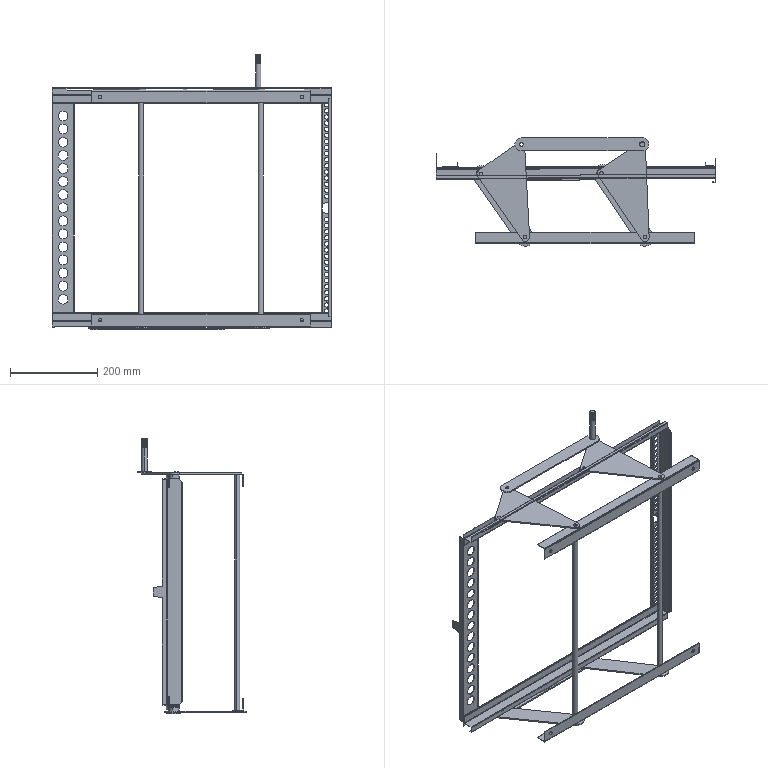Assembly | SolidWorks | mm | 22 component files | 22 solids | 557 faces | box 641.35 x 247.6 x 631 mm | volume 593883 mm3 | cylinder 298 | plane 246 | cone 10 | spline 3 | commonest cylinder face diameters 10 x72 8 x60 12 x46 22 x38 1.473 x20 3.473 x18 12.5 x16 30 x6
Bill of materials:
40 MM KOL | 2 |  | Flat, thin, straight link plate with fully rounded (obround) ends and one small through-hole near each end.
ALK K_EBENT | 2 |  | Straight equal-or-near-equal leg angle (L-section) bar with a rounded inner bend; each leg has two through-holes.
DEM_R TEKER | 4 |  | Short thick cylindrical ring/spacer with a central through-bore and a chamfer on one outer bottom edge.
gen par_a | 2 |  | Flat thin triangular plate (gusset-like outline) with rounded corners and a through-hole at each of the three corners.
I KOL | 1 |  | Long flat thin bar with rounded (obround) ends and one small through-hole near each end; slender relative to unnamed part.
M_LL_ KOL | 1 |  | Flat obround bar with a through-hole at one end and a perpendicular cylindrical pin standing from the other end; the pin's outer portion carries thread-like ridges and the base shows a disc/flange at the plate.
ORTA M_L | 2 |  | Long slender solid cylindrical rod with short slightly reduced-diameter stepped ends.
PER_N | 4 |  | Solid stepped cylinder: a larger-diameter base with a coaxial smaller-diameter boss on top.
RAY SA | 1 |  | Long formed sheet-metal profile with a multi-bend section: a C/hooked return on one side, a horizontal web, and a tall U-shaped double-wall fold on the other side; small notches/cut-outs along one lower edge.
RAY SOL | 1 |  | Long formed sheet-metal profile similar in section to unnamed part but mirrored/inverted, with the U-fold downward and the C-return upward; long slots run along one flange.
tepsi _st dayama delikli | 1 |  | Sheet-metal U-channel (wide web, two flanges of unequal height) with a single row of evenly spaced round holes along the web and a small tab protruding from one face near mid-length.
tepsi _st kademeli | 1 |  | Long slender formed sheet-metal post with a multi-bend section (offset flanges and a hooked lip), a dense row of round holes along one face, a punched tab/lance near mid-length, and angled corners at the ends.
Mates:
1. coincident | gen par_a-1 face at (-45.148, 24.677, 186.974) dir (0, 0, 1) | M_LL_ KOL-1 face at (-53.921, 237.176, 186.974) dir (0, 0, -1)
2. concentric | M_LL_ KOL-1 face at (223.079, 237.279, 186.974) dir (0, 0, 1) r 4 | gen par_a-2 face at (223.079, 237.279, 183.974) dir (0, 0, 1) r 4
3. coincident | gen par_a-2 face at (228.852, 24.677, 183.974) dir (0, 0, -1) | ALK K_EBENT-1 face at (341.852, 11.677, 183.974) dir (0, 0, 1)
4. concentric | gen par_a-2 face at (228.852, 24.677, 183.974) dir (0, 0, 1) r 4 | ALK K_EBENT-1 face at (228.852, 24.677, 173.974) dir (0, 0, 1) r 5
5. concentric | gen par_a-1 face at (-45.148, 24.677, 183.974) dir (0, 0, 1) r 4 | ALK K_EBENT-1 face at (-45.148, 24.677, 173.974) dir (0, 0, 1) r 5
6. parallel | ALK K_EBENT-1 face at (341.852, 10.177, 182.474) dir (0, -1, 0) | assembly plane at (0, 0, 0) dir (0, 1, 0)
7. coincident | gen par_a-2 face at (228.852, 24.677, 183.974) dir (0, 0, 1) r 4 | ORTA M_L-2 edge at (228.852, 24.677, 187.474) dir (0, 0, 1) r 4
8. coincident | ALK K_EBENT-1 face at (341.852, 11.677, 182.474) dir (0, 0, -1) | ORTA M_L-2 edge at (228.852, 24.677, 182.474) dir (0, 0, 1) r 6
9. concentric | ALK K_EBENT-1 face at (-45.148, 24.677, 173.974) dir (0, 0, 1) r 5 | ORTA M_L-1 face at (-45.148, 24.677, 187.474) dir (0, 0, -1) r 4
10. coincident | ALK K_EBENT-1 face at (341.852, 11.677, 182.474) dir (0, 0, -1) | ORTA M_L-1 face at (-45.148, 24.677, 182.474) dir (0, 0, 1)
11. concentric | ORTA M_L-2 edge at (228.852, 24.677, -362.526) dir (0, 0, -1) r 4 | ALK K_EBENT-3 edge at (228.852, 24.677, -359.026) dir (0, 0, -1) r 5
12. concentric | ORTA M_L-1 face at (-45.148, 24.677, -362.526) dir (0, 0, 1) r 4 | ALK K_EBENT-3 edge at (-45.148, 24.677, -359.026) dir (0, 0, -1) r 5
13. coincident | ORTA M_L-2 edge at (228.852, 24.677, -357.526) dir (0, 0, 1) r 6 | ALK K_EBENT-3 face at (-158.148, 11.677, -357.526) dir (0, 0, 1)
14. coincident | ORTA M_L-1 face at (-45.148, 24.677, -357.526) dir (0, 0, -1) | ALK K_EBENT-3 face at (-158.148, 11.677, -357.526) dir (0, 0, 1)
15. coincident | ALK K_EBENT-3 face at (-158.148, 11.677, -359.026) dir (0, 0, -1) | 40 MM KOL-1 face at (228.852, 24.677, -359.026) dir (0, 0, 1)
16. coincident | gen par_a-1 face at (-45.148, 24.677, 183.974) dir (0, 0, -1) | ALK K_EBENT-1 face at (341.852, 11.677, 183.974) dir (0, 0, 1)
17. concentric | DEM_R TEKER-1 face at (-146.473, 169.805, 180.974) dir (0, 0, -1) r 6.25 | PER_N-1 face at (-146.473, 169.805, 180.974) dir (0, 0, -1) r 6.25
18. coincident | DEM_R TEKER-1 face at (-146.473, 169.805, 173.974) dir (0, 0, -1) | PER_N-1 face at (-146.473, 169.805, 173.974) dir (0, 0, -1)
19. concentric | gen par_a-1 face at (-146.473, 169.805, 183.974) dir (0, 0, 1) r 4 | PER_N-1 face at (-146.473, 169.805, 186.974) dir (0, 0, -1) r 4
20. coincident | gen par_a-1 face at (-45.148, 24.677, 183.974) dir (0, 0, -1) | DEM_R TEKER-1 face at (-146.473, 169.805, 183.974) dir (0, 0, 1)
21. concentric | DEM_R TEKER-3 face at (129.585, 171.221, 183.974) dir (0, 0, -1) r 4 | PER_N-2 face at (129.585, 171.221, 186.974) dir (0, 0, -1) r 4
22. coincident | DEM_R TEKER-3 face at (129.585, 171.221, 173.974) dir (0, 0, -1) | PER_N-2 face at (129.585, 171.221, 173.974) dir (0, 0, -1)
23. concentric | gen par_a-2 face at (129.585, 171.221, 183.974) dir (0, 0, 1) r 4 | PER_N-2 face at (129.585, 171.221, 186.974) dir (0, 0, -1) r 4
24. coincident | gen par_a-2 face at (228.852, 24.677, 183.974) dir (0, 0, -1) | DEM_R TEKER-3 face at (129.585, 171.221, 183.974) dir (0, 0, 1)
25. concentric | PER_N-4 face at (130.519, 171.849, -356.026) dir (0, 0, 1) r 6.25 | DEM_R TEKER-5 face at (130.519, 171.849, -356.026) dir (0, 0, 1) r 6.25
26. coincident | PER_N-4 face at (130.519, 171.849, -349.026) dir (0, 0, 1) | DEM_R TEKER-5 face at (130.519, 171.849, -349.026) dir (0, 0, 1)
27. concentric | 40 MM KOL-1 face at (130.519, 171.849, -362.026) dir (0, 0, 1) r 4 | PER_N-4 face at (130.519, 171.849, -362.026) dir (0, 0, 1) r 4
28. coincident | 40 MM KOL-1 face at (228.852, 24.677, -359.026) dir (0, 0, 1) | DEM_R TEKER-5 face at (130.519, 171.849, -359.026) dir (0, 0, -1)
29. coincident | ALK K_EBENT-3 face at (-158.148, 11.677, -359.026) dir (0, 0, -1) | 40 MM KOL-3 face at (-45.148, 24.677, -359.026) dir (0, 0, 1)
30. concentric | gen par_a-1 face at (-53.921, 237.176, 183.974) dir (0, 0, 1) r 4 | M_LL_ KOL-1 face at (-53.921, 237.176, 186.974) dir (0, 0, 1) r 4
31. concentric | 40 MM KOL-3 face at (-146.473, 169.805, -362.026) dir (0, 0, 1) r 4 | DEM_R TEKER-1 face at (-146.473, 169.805, 173.974) dir (0, 0, 1) r 11
32. coincident | 40 MM KOL-3 face at (-45.148, 24.677, -362.026) dir (0, 0, -1) | I KOL-1 face at (-146.473, 169.805, -362.026) dir (0, 0, 1)
33. concentric | 40 MM KOL-3 face at (-146.473, 169.805, -362.026) dir (0, 0, 1) r 4 | I KOL-1 face at (-146.473, 169.805, -365.026) dir (0, 0, 1) r 4
34. coincident | PER_N-4 edge at (130.519, 171.849, -362.026) dir (0, 0, -1) r 4 | I KOL-1 face at (130.519, 171.849, -365.026) dir (0, 0, 1) r 4
35. concentric | DEM_R TEKER-6 face at (-146.473, 169.805, -356.026) dir (0, 0, 1) r 6.25 | PER_N-5 face at (-146.473, 169.805, -356.026) dir (0, 0, 1) r 6.25
36. coincident | DEM_R TEKER-6 face at (-146.473, 169.805, -349.026) dir (0, 0, 1) | PER_N-5 face at (-146.473, 169.805, -349.026) dir (0, 0, 1)
37. concentric | 40 MM KOL-3 face at (-146.473, 169.805, -362.026) dir (0, 0, 1) r 4 | PER_N-5 face at (-146.473, 169.805, -362.026) dir (0, 0, 1) r 4
38. coincident | 40 MM KOL-3 face at (-45.148, 24.677, -359.026) dir (0, 0, 1) | DEM_R TEKER-6 face at (-146.473, 169.805, -359.026) dir (0, 0, -1)
39. tangent | DEM_R TEKER-1 face at (-146.473, 169.805, 173.974) dir (0, 0, 1) r 11 | RAY MONTAJ-1/RAY SOL-2 face at (390.845, 161.561, 187.974) dir (-0.005128, 1, 0)
40. tangent | DEM_R TEKER-3 face at (129.585, 171.221, 173.974) dir (0, 0, 1) r 11 | RAY MONTAJ-1/RAY SOL-2 face at (390.845, 161.561, 187.974) dir (-0.005128, 1, 0)
41. coincident | DEM_R TEKER-1 face at (-146.473, 169.805, 173.974) dir (0, 0, -1) | RAY MONTAJ-1/RAY SOL-2 face at (390.845, 161.561, 173.974) dir (0, 0, 1)
42. tangent | DEM_R TEKER-6 face at (-146.473, 169.805, -349.026) dir (0, 0, -1) r 11 | RAY MONTAJ-1/RAY SA-2 face at (-249.146, 158.279, -360.026) dir (-0.005128, 1, 0)
43. concentric | ALK K_EBENT-3 face at (228.852, 24.677, -349.026) dir (0, 0, -1) r 5 | 40 MM KOL-1 face at (228.852, 24.677, -362.026) dir (0, 0, 1) r 4
44. concentric | ALK K_EBENT-3 face at (-45.148, 24.677, -349.026) dir (0, 0, -1) r 5 | 40 MM KOL-3 face at (-45.148, 24.677, -362.026) dir (0, 0, 1) r 4
45. coincident | tepsi _st kademeli-1 face at (324.996, 68.699, -25.448) dir (0, 1, 0) | RAY SA-2 face at (825.996, 68.699, 592.552) dir (0, -1, 0)
46. coincident | tepsi _st kademeli-1 face at (324.996, 67.699, -47.448) dir (0, 0, 1) | RAY SA-2 face at (843.259, 72.699, -47.448) dir (0, 0, -1)
47. coincident | tepsi _st kademeli-1 face at (844.996, 69.436, -46.712) dir (1, 0, 0) | RAY SA-2 face at (844.996, 94.699, 592.552) dir (1, 0, 0)
48. coincident | tepsi _st dayama delikli-1 face at (842.496, 68.699, 542.552) dir (0, 1, 0) | RAY SA-2 face at (825.996, 68.699, 592.552) dir (0, -1, 0)
49. coincident | RAY SA-2 face at (844.996, 72.699, 592.552) dir (0, 1, 0) | RAY SOL-2 face at (324.996, 72.699, -47.448) dir (0, 1, 0)
50. coincident | RAY SA-2 face at (845.733, 95.699, 592.552) dir (0, 0, 1) | RAY SOL-2 face at (326.733, 72.699, 592.552) dir (0, 0, 1)
51. coincident | tepsi _st kademeli-1 face at (324.996, 68.699, -46.712) dir (-1, 0, 0) | RAY SOL-2 face at (324.996, 94.699, -47.448) dir (-1, 0, 0)
52. coincident | tepsi _st dayama delikli-1 face at (842.496, 68.699, 592.552) dir (0, 0, 1) | RAY SOL-2 face at (326.733, 72.699, 592.552) dir (0, 0, 1)
53. width | RAY SOL-2 face at (316.496, 69.699, -47.448) dir (-1, 0, 0) | RAY SA-2 face at (853.496, 69.699, 592.552) dir (1, 0, 0) | tepsi _st dayama delikli-1 face at (842.496, 66.963, 591.552) dir (1, 0, 0) | tepsi _st dayama delikli-1 face at (327.496, 66.963, 543.552) dir (-1, 0, 0)